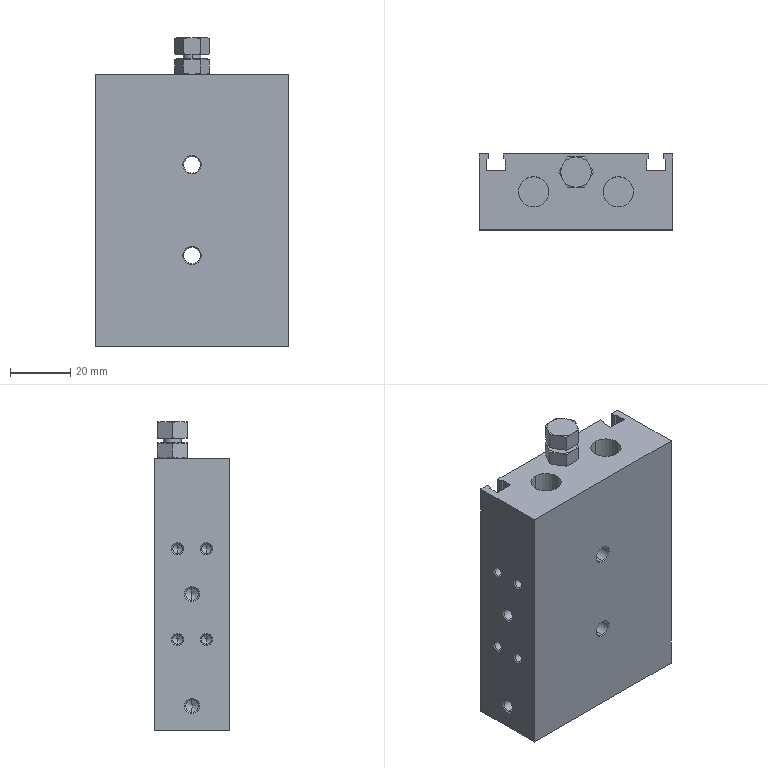Component | SolidWorks | CXSM20-20-Z73(0_0_0)-1_CXSM20-20(0_0)_BODY-1 | 1 solid | 161 faces | box 64 x 25 x 102 mm | volume 116436 mm3 | cone 76 | plane 43 | cylinder 42 | commonest cylinder face diameters 3.242 x16 4.134 x8 9.5 x4 20 x4 10 x4 5.5 x4 6 x2
build123d program:
from build123d import *

# Parameters (mm, degrees)
BOSS_EXTRUDE1_DEPTH = 90
SKETCH22_R          = 11
CUT_EXTRUDE1_DEPTH  = 12


with BuildPart() as part:
    # Sketch1 → Boss-Extrude1 (new body)
    with BuildSketch(Plane.XY):
        Polygon((-12.5, 32), (-12.5, -32), (12.5, -32), (12.5, -29), (11.075, -29), (10.7, -29.65), (7.1, -29.65), (7.1, -23.35), (10.7, -23.35), (11.075, -24), (12.5, -24), (12.5, 24), (11.075, 24), (10.7, 23.35), (7.1, 23.35), (7.1, 29.65), (10.7, 29.65), (11.075, 29), (12.5, 29), (12.5, 32), align=None)
    extrude(amount=-BOSS_EXTRUDE1_DEPTH)

    # Sketch2 → Cut-Revolve1 (revolve, cut)
    with BuildSketch(Plane(origin=(0, 0, 0), x_dir=(0, 0, -1), z_dir=(1, 0, 0)), mode=Mode.PRIVATE) as cut_revolve1_sk:
        Polygon((0, 14), (0, 19), (30, 19), (30, 24), (55, 24), (55, 14), align=None)
    revolve(cut_revolve1_sk.sketch.rotate(Axis((0, 14, -55), (0, 0, 1)), 270), axis=Axis((0, 14, -55), (0, 0, 1)), mode=Mode.SUBTRACT)

    # Sketch3 → Cut-Revolve2 (revolve, cut)
    with BuildSketch(Plane(origin=(0, 0, 0), x_dir=(0, 0, -1), z_dir=(1, 0, 0)), mode=Mode.PRIVATE) as cut_revolve2_sk:
        Polygon((0, -14), (0, -9), (30, -9), (30, -4), (55, -4), (55, -14), align=None)
    revolve(cut_revolve2_sk.sketch.rotate(Axis((0, -14, -55), (0, 0, 1)), 270), axis=Axis((0, -14, -55), (0, 0, 1)), mode=Mode.SUBTRACT)

    # Sketch4 → Cut-Revolve3 (revolve, cut)
    with BuildSketch(Plane.XY.offset(-30), mode=Mode.PRIVATE) as cut_revolve3_sk:
        Polygon((-12.5, 0), (-12.5, 2.75), (7.2, 2.75), (7.2, 4.75), (12.5, 4.75), (12.5, 0), align=None)
    revolve(cut_revolve3_sk.sketch.rotate(Axis((12.5, 0, -30), (-1, 0, 0)), 270), axis=Axis((12.5, 0, -30), (-1, 0, 0)), mode=Mode.SUBTRACT)

    # Sketch5 → Cut-Revolve4 (revolve, cut)
    with BuildSketch(Plane.XY.offset(-60), mode=Mode.PRIVATE) as cut_revolve4_sk:
        Polygon((-12.5, 0), (-12.5, 2.75), (7.2, 2.75), (7.2, 4.75), (12.5, 4.75), (12.5, 0), align=None)
    revolve(cut_revolve4_sk.sketch.rotate(Axis((12.5, 0, -60), (-1, 0, 0)), 270), axis=Axis((12.5, 0, -60), (-1, 0, 0)), mode=Mode.SUBTRACT)

    # Sketch6 → Cut-Revolve5 (revolve, cut)
    with BuildSketch(Plane.XY.offset(-30), mode=Mode.PRIVATE) as cut_revolve5_sk:
        Polygon((-12.5, 0), (-12.5, 3), (-11.959, 2.458), (-2.5, 2.458), (-1.081, 0), align=None)
    revolve(cut_revolve5_sk.sketch.rotate(Axis((-1.081, 0, -30), (-1, 0, 0)), 270), axis=Axis((-1.081, 0, -30), (-1, 0, 0)), mode=Mode.SUBTRACT)

    # Sketch7 → Cut-Revolve6 (revolve, cut)
    with BuildSketch(Plane.XY.offset(-60), mode=Mode.PRIVATE) as cut_revolve6_sk:
        Polygon((-12.5, 0), (-12.5, 3), (-11.959, 2.458), (-2.5, 2.458), (-1.081, 0), align=None)
    revolve(cut_revolve6_sk.sketch.rotate(Axis((-1.081, 0, -60), (-1, 0, 0)), 270), axis=Axis((-1.081, 0, -60), (-1, 0, 0)), mode=Mode.SUBTRACT)

    # Sketch8 → Cut-Revolve7 (revolve, cut)
    with BuildSketch(Plane(origin=(0, 0, 0), x_dir=(0, 0, -1), z_dir=(1, 0, 0)), mode=Mode.PRIVATE) as cut_revolve7_sk:
        Polygon((45, 26.307), (42.933, 27.5), (42.933, 31.567), (42.5, 32), (45, 32), align=None)
    revolve(cut_revolve7_sk.sketch.rotate(Axis((0, 32, -45), (0, -1, 0)), 180), axis=Axis((0, 32, -45), (0, -1, 0)), mode=Mode.SUBTRACT)

    # Sketch9 → Cut-Revolve8 (revolve, cut)
    with BuildSketch(Plane(origin=(0, 0, 0), x_dir=(0, 0, -1), z_dir=(1, 0, 0)), mode=Mode.PRIVATE) as cut_revolve8_sk:
        Polygon((82, 26.307), (79.933, 27.5), (79.933, 31.567), (79.5, 32), (82, 32), align=None)
    revolve(cut_revolve8_sk.sketch.rotate(Axis((0, 32, -82), (0, -1, 0)), 180), axis=Axis((0, 32, -82), (0, -1, 0)), mode=Mode.SUBTRACT)

    # Sketch10 → Cut-Revolve9 (revolve, cut)
    with BuildSketch(Plane(origin=(0, 0, 0), x_dir=(0, 0, -1), z_dir=(1, 0, 0)), mode=Mode.PRIVATE) as cut_revolve9_sk:
        Polygon((45, -32), (42.5, -32), (42.933, -31.567), (42.933, -27.5), (45, -26.307), align=None)
    revolve(cut_revolve9_sk.sketch.rotate(Axis((0, -26.307, -45), (0, -1, 0)), 180), axis=Axis((0, -26.307, -45), (0, -1, 0)), mode=Mode.SUBTRACT)

    # Sketch11 → Cut-Revolve10 (revolve, cut)
    with BuildSketch(Plane(origin=(0, 0, 0), x_dir=(0, 0, -1), z_dir=(1, 0, 0)), mode=Mode.PRIVATE) as cut_revolve10_sk:
        Polygon((82, -32), (79.5, -32), (79.933, -31.567), (79.933, -27.5), (82, -26.307), align=None)
    revolve(cut_revolve10_sk.sketch.rotate(Axis((0, -26.307, -82), (0, -1, 0)), 180), axis=Axis((0, -26.307, -82), (0, -1, 0)), mode=Mode.SUBTRACT)

    # Sketch12 → Cut-Revolve11 (revolve, cut)
    with BuildSketch(Plane.XY.offset(-30), mode=Mode.PRIVATE) as cut_revolve11_sk:
        Polygon((-4.75, 25.564), (-6.371, 26.5), (-6.371, 31.621), (-6.75, 32), (-4.75, 32), align=None)
    revolve(cut_revolve11_sk.sketch.rotate(Axis((-4.75, 32, -30), (0, -1, 0)), 90), axis=Axis((-4.75, 32, -30), (0, -1, 0)), mode=Mode.SUBTRACT)

    # Sketch13 → Cut-Revolve12 (revolve, cut)
    with BuildSketch(Plane.XY.offset(-30), mode=Mode.PRIVATE) as cut_revolve12_sk:
        Polygon((4.75, -32), (2.75, -32), (3.129, -31.621), (3.129, -26.5), (4.75, -25.564), align=None)
    revolve(cut_revolve12_sk.sketch.rotate(Axis((4.75, -25.564, -30), (0, -1, 0)), 90), axis=Axis((4.75, -25.564, -30), (0, -1, 0)), mode=Mode.SUBTRACT)

    # Sketch14 → Cut-Revolve13 (revolve, cut)
    with BuildSketch(Plane.XY.offset(-60), mode=Mode.PRIVATE) as cut_revolve13_sk:
        Polygon((4.75, 25.564), (3.129, 26.5), (3.129, 31.621), (2.75, 32), (4.75, 32), align=None)
    revolve(cut_revolve13_sk.sketch.rotate(Axis((4.75, 32, -60), (0, -1, 0)), 90), axis=Axis((4.75, 32, -60), (0, -1, 0)), mode=Mode.SUBTRACT)

    # Sketch15 → Cut-Revolve14 (revolve, cut)
    with BuildSketch(Plane.XY.offset(-60), mode=Mode.PRIVATE) as cut_revolve14_sk:
        Polygon((-4.75, 25.564), (-6.371, 26.5), (-6.371, 31.621), (-6.75, 32), (-4.75, 32), align=None)
    revolve(cut_revolve14_sk.sketch.rotate(Axis((-4.75, 32, -60), (0, -1, 0)), 90), axis=Axis((-4.75, 32, -60), (0, -1, 0)), mode=Mode.SUBTRACT)

    # Sketch16 → Cut-Revolve15 (revolve, cut)
    with BuildSketch(Plane.XY.offset(-30), mode=Mode.PRIVATE) as cut_revolve15_sk:
        Polygon((4.75, 25.564), (3.129, 26.5), (3.129, 31.621), (2.75, 32), (4.75, 32), align=None)
    revolve(cut_revolve15_sk.sketch.rotate(Axis((4.75, 32, -30), (0, -1, 0)), 90), axis=Axis((4.75, 32, -30), (0, -1, 0)), mode=Mode.SUBTRACT)

    # Sketch17 → Cut-Revolve16 (revolve, cut)
    with BuildSketch(Plane.XY.offset(-60), mode=Mode.PRIVATE) as cut_revolve16_sk:
        Polygon((-4.75, -32), (-6.75, -32), (-6.371, -31.621), (-6.371, -26.5), (-4.75, -25.564), align=None)
    revolve(cut_revolve16_sk.sketch.rotate(Axis((-4.75, -25.564, -60), (0, -1, 0)), 90), axis=Axis((-4.75, -25.564, -60), (0, -1, 0)), mode=Mode.SUBTRACT)

    # Sketch18 → Cut-Revolve17 (revolve, cut)
    with BuildSketch(Plane.XY.offset(-60), mode=Mode.PRIVATE) as cut_revolve17_sk:
        Polygon((4.75, -32), (2.75, -32), (3.129, -31.621), (3.129, -26.5), (4.75, -25.564), align=None)
    revolve(cut_revolve17_sk.sketch.rotate(Axis((4.75, -25.564, -60), (0, -1, 0)), 90), axis=Axis((4.75, -25.564, -60), (0, -1, 0)), mode=Mode.SUBTRACT)

    # Sketch19 → Cut-Revolve18 (revolve, cut)
    with BuildSketch(Plane.XY.offset(-30), mode=Mode.PRIVATE) as cut_revolve18_sk:
        Polygon((-4.75, -32), (-6.75, -32), (-6.371, -31.621), (-6.371, -26.5), (-4.75, -25.564), align=None)
    revolve(cut_revolve18_sk.sketch.rotate(Axis((-4.75, -25.564, -30), (0, -1, 0)), 90), axis=Axis((-4.75, -25.564, -30), (0, -1, 0)), mode=Mode.SUBTRACT)

    # Sketch20 → Revolve1 (revolve)
    with BuildSketch(Plane(origin=(6.5, 0, 0), x_dir=(0, 0, -1), z_dir=(1, 0, 0)), mode=Mode.PRIVATE) as revolve1_sk:
        Polygon((-5, 0), (-5, 5), (-3.66, 10), (-1.34, 10), (0, 5), (0, 0), align=None)
    revolve(revolve1_sk.sketch.rotate(Axis((6.5, 0, 0), (0, 0, 1)), 270), axis=Axis((6.5, 0, 0), (0, 0, 1)))

    # Sketch21 → Revolve2 (revolve)
    with BuildSketch(Plane(origin=(6.5, 0, 0), x_dir=(0, 0, -1), z_dir=(1, 0, 0)), mode=Mode.PRIVATE) as revolve2_sk:
        Polygon((-12, 0), (-12, 5), (-10.66, 10), (-7.84, 10), (-6.5, 5), (-6.5, 3), (-5, 3), (-5, 0), align=None)
    revolve(revolve2_sk.sketch.rotate(Axis((6.5, 0, 5), (0, 0, 1)), 270), axis=Axis((6.5, 0, 5), (0, 0, 1)))

    # Sketch22 → Cut-Extrude1 (cut)
    with BuildSketch(Plane.XY):
        with Locations((6.5, 0)):
            Circle(SKETCH22_R)
        Polygon((1.5, 2.887), (1.5, -2.887), (6.5, -5.774), (11.5, -2.887), (11.5, 2.887), (6.5, 5.774), align=None, mode=Mode.SUBTRACT)
    extrude(amount=CUT_EXTRUDE1_DEPTH, mode=Mode.SUBTRACT)


solid = part.part

# Placed as in the assembly
solid = solid.moved(Location((955.263, 384.593, -356.196), (0, 0, 90)))